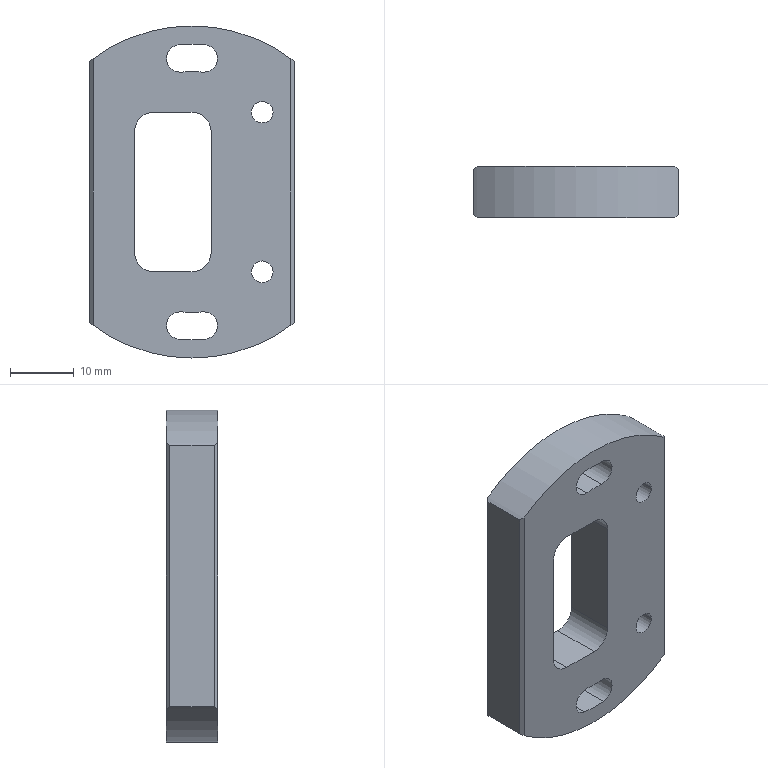CAM job | Mastercam | mm | 13 operations | part box 32 x 8 x 52
1. Facing | 24 - 100 平铣刀
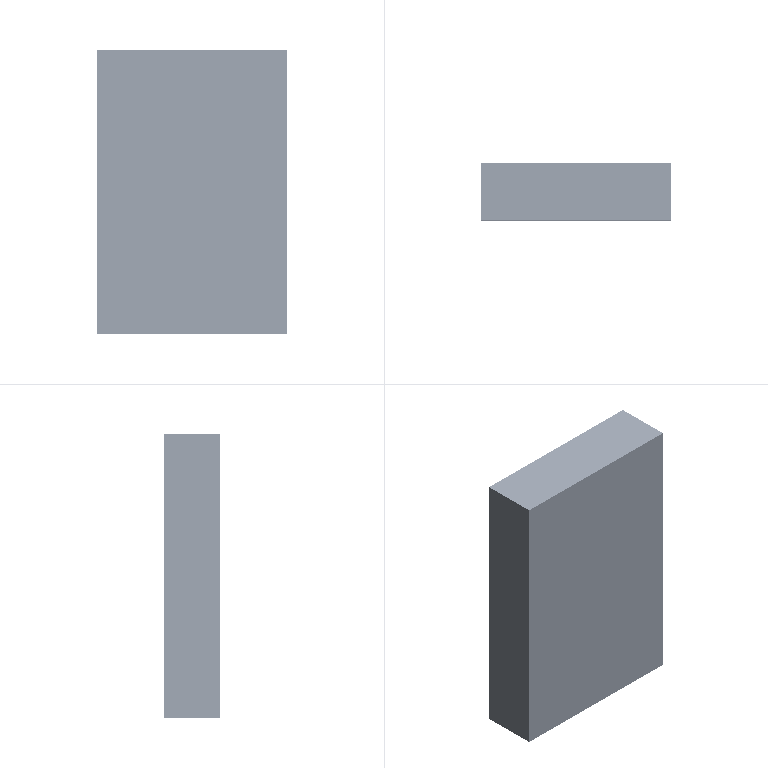2. Contour (Ramp) | 10 - 10 平铣刀
3. Contour (Ramp) | 6 - 6 平铣刀
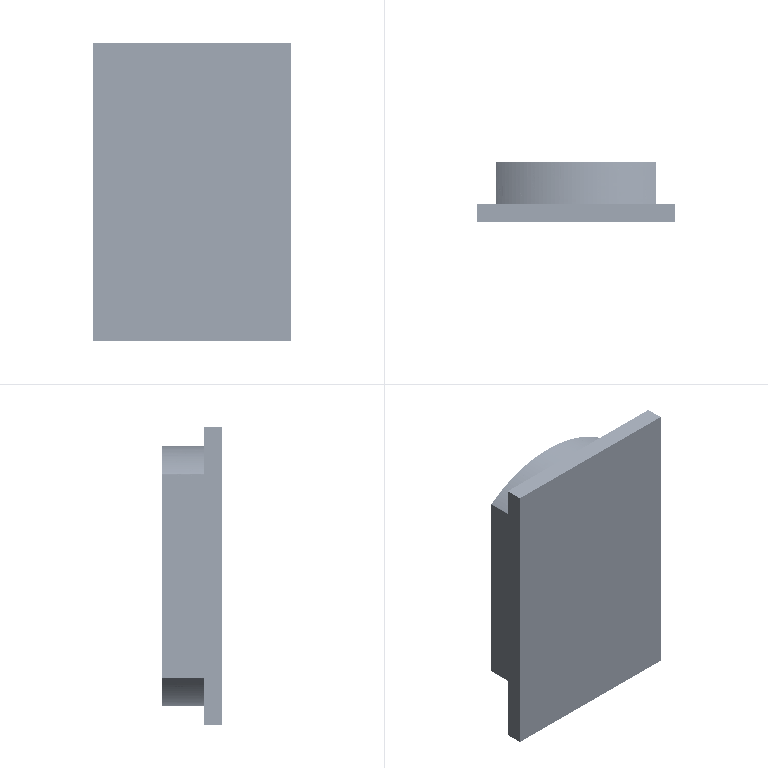4. Contour (2D) | 6 - 6 平铣刀
5. Contour (Ramp) | 3 - 3 平铣刀
6. Contour (Ramp) | 3 - 3 平铣刀
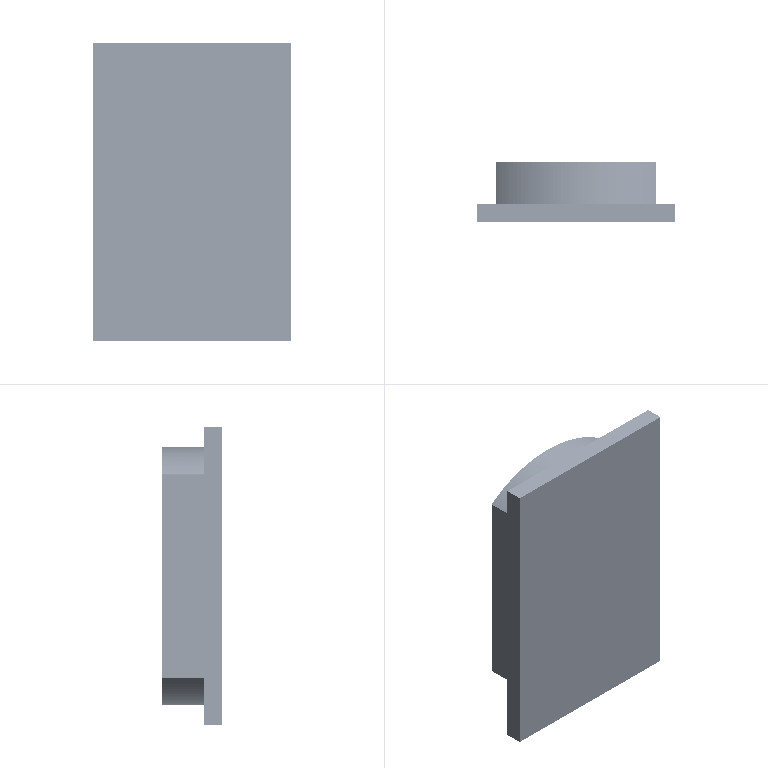7. Contour (Ramp) | 3 - 3 平铣刀
8. Contour (2D chamfer) | 7 - 4 倒角刀
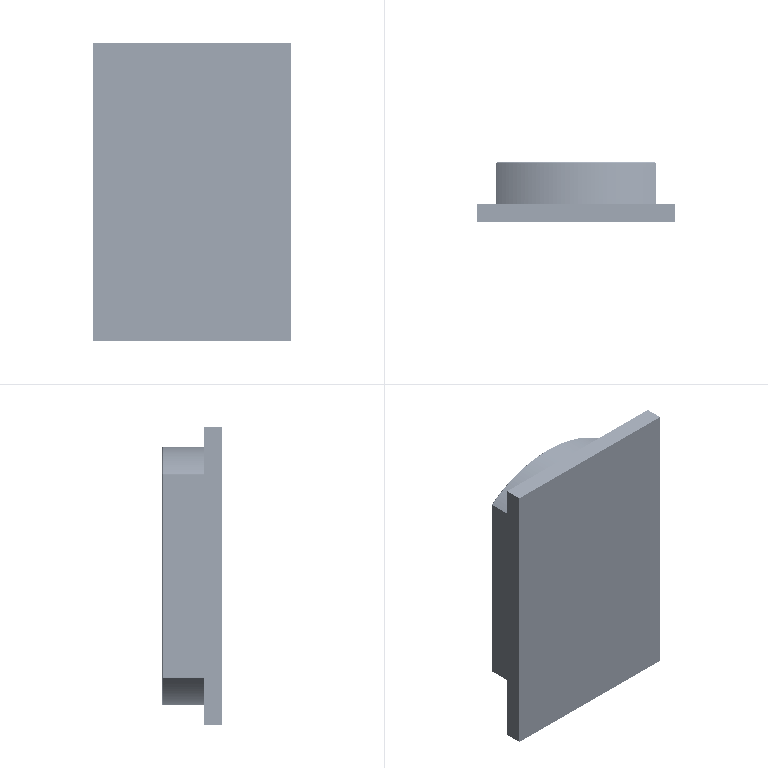9. Contour (2D chamfer) | 7 - 4 倒角刀
10. Facing | 24 - 100 平铣刀
11. Contour (2D chamfer) | 7 - 4 倒角刀
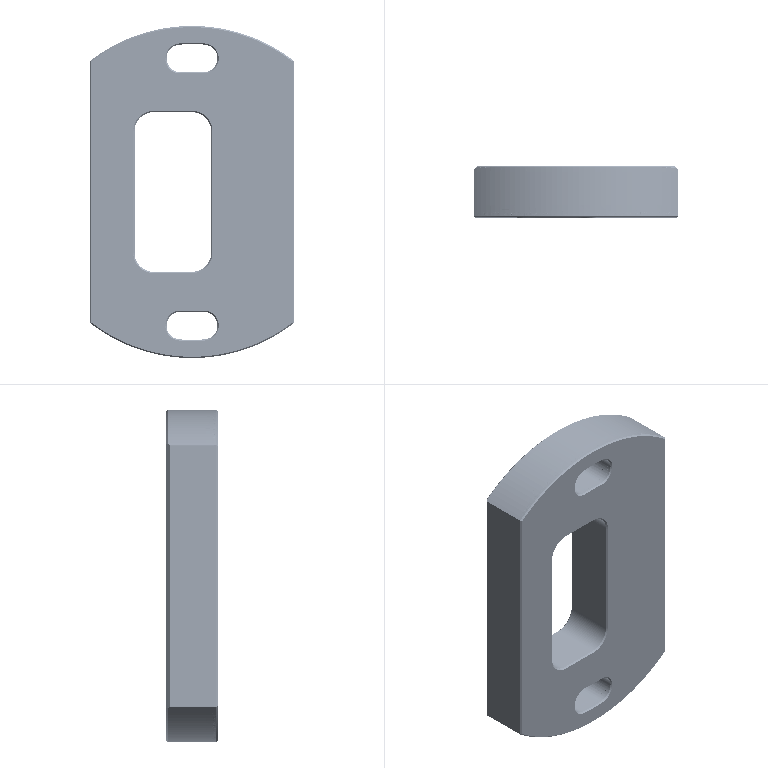12. Contour (2D chamfer) | 7 - 4 倒角刀
13. Drill/Counterbore | 7 - 4 倒角刀